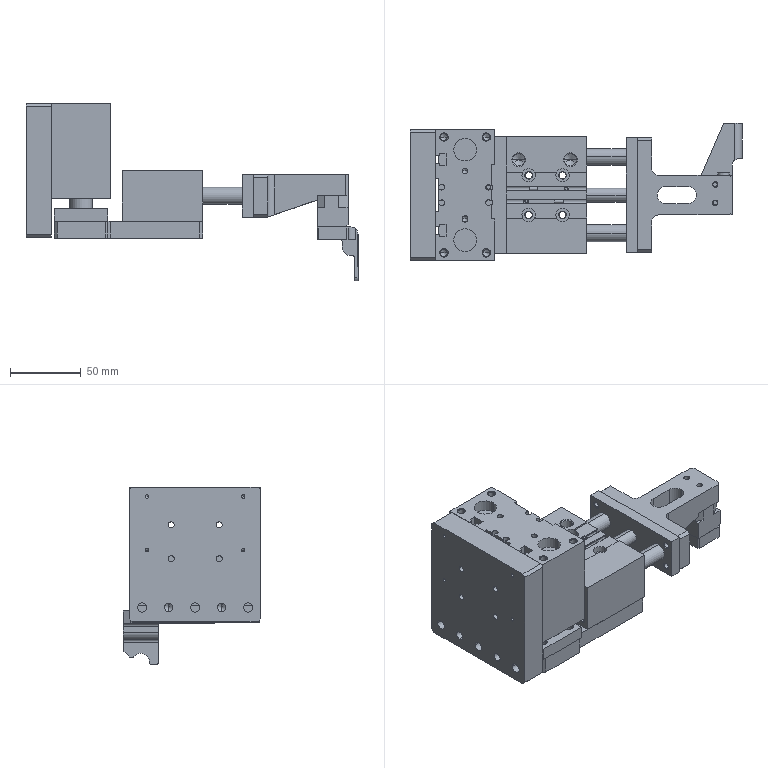Assembly | SolidWorks | mm | 19 component files | 19 solids | 919 faces | box 235 x 97.5 x 125.5 mm | volume 753632 mm3 | cylinder 362 | plane 357 | cone 184 | torus 16 | commonest cylinder face diameters 4 x40 4.917 x32 3 x26 6 x24 8.566 x24 11 x22 6.6 x22 2.5 x16
Bill of materials:
AX.B92.SA.7371.18 | 1 | 6061 | Flat rectangular plate with a wider stepped section at one end, chamfered corners, and a pattern of through holes of three sizes.
AX.B92.SA.7371.20 | 1 | 6061 | T-shaped bracket: a flat arm with an elongated slot and two small holes, joined to a perpendicular mounting flange that has four holes. A tapered web sits under the arm.
AX.B92.SA.7371.25 | 1 | 7075 | Thick square-ish plate with chamfered corners, four small holes in a square pattern, and three larger holes in a row along one edge.
AX.B92.SA.7371.37 | 1 | 40Cr | L-shaped bracket: a flat horizontal arm with two counterbored holes, joined to a downward leg with a rounded outer corner. The leg ends in a semicircular notch.
SCHUNK-0303022 | 2 | 1.231 (40CrMnMoS8-6) | Revolved part with a cylindrical head containing a hexagonal socket, an hourglass-shaped neck groove, a larger cylindrical body, and a smaller end spigot.
D_M9P_MGP_Z_6 | 4 |  | Stepped cylindrical shaft with a smaller pilot end and a long main section that has one wide flat machined along its length.
MGP_Z_PLUG_20_9 | 2 |  | Plain solid cylinder with flat ends and no visible holes, chamfers, or other features.
MGPM20_20Z_0_BODY_2 | 1 |  | Rectangular block with two parallel longitudinal grooves on top, several counterbored or stepped holes, two large cross-bores through the end faces, and T-shaped slots and small round grooves on the bottom.
MGPM20_20Z_0_ROD_4 | 1 |  | Rectangular flange plate with four corner holes and two small central holes, and three parallel round rods sticking out from one face. The middle rod is shorter and has a disc-shaped head.
MGP_Z_PLUG_25_9 | 2 |  | Plain solid cylinder with flat ends and no visible holes, chamfers, or other features. It looks the same as unnamed part.
MGPM25_30Z_0_BODY_2 | 1 |  | Rectangular block with two large vertical through bores, small countersunk holes at the corners, T-shaped slots and semicircular notches along the sides, two parallel vertical grooves on one face, and several side holes.
MGPM25_30Z_0_ROD_4 | 1 |  | Rectangular base plate with four corner holes and three upright cylindrical posts in a row. The middle post is shorter, thinner, and capped with a larger disc.
SCHUNK-0303023 BSWS-B 64 | 1 | Q235-A | Roughly rectangular prismatic block with a stepped, angled notch cut into one vertical corner. Two parallel cylindrical pins with chamfered tips stick up from the top face, and each pin sits in a shallow annular recess. A further short cylindrical boss appears to stick out from a side face that is hidden in the isometric view.
Mates:
1. coincident | AX.B92.SA.7371.25-2 face at (-0.5788, 7.188, 28.472) dir (1, 0, 0) | MGPM25-30Z-M9P-1/MGPM25_30Z_0_BODY_2-1 face at (-0.5788, 65.688, 123.472) dir (-1, 0, 0)
2. width | MGPM25-30Z-M9P-1/MGPM25_30Z_0_BODY_2-1 face at (-0.5788, 100.188, 123.472) dir (0, 1, 0) | MGPM25-30Z-M9P-1/MGPM25_30Z_0_BODY_2-1 face at (41.421, 7.188, 123.472) dir (0, -1, 0) | AX.B92.SA.7371.25-2 face at (-9.579, 100.188, 75.972) dir (0, 1, 0) | AX.B92.SA.7371.25-2 face at (-9.579, 7.188, 75.972) dir (0, -1, 0)
3. coincident | AX.B92.SA.7371.25-2 face at (-0.5788, 7.188, 123.472) dir (0, 0, 1) | MGPM25-30Z-M9P-1/MGPM25_30Z_0_BODY_2-1 face at (36.921, 59.188, 123.472) dir (0, 0, 1)
4. coincident | AX.B92.SA.7371.18-2 face at (53.921, 53.688, 39.972) dir (0, 0, 1) | MGPM25-30Z-M9P-1/MGPM25_30Z_0_ROD_4-1 face at (20.421, 53.688, 39.972) dir (0, 0, -1)
5. concentric | AX.B92.SA.7371.18-2 face at (7.421, 92.688, 27.972) dir (0, 0, -1) r 5.5 | MGPM25-30Z-M9P-1/MGPM25_30Z_0_ROD_4-1 face at (7.421, 92.688, 39.972) dir (0, 0, 1) r 2.458
6. parallel | AX.B92.SA.7371.18-2 face at (106.421, 99.188, 39.972) dir (0, 1, 0) | MGPM25-30Z-M9P-1/MGPM25_30Z_0_ROD_4-1 face at (1.421, 99.188, 48.972) dir (0, 1, 0)
7. concentric | AX.B92.SA.7371.18-2 face at (65.421, 67.688, 27.972) dir (0, 0, -1) r 5.5 | MGPM20-20Z-M9P-1/MGPM20_20Z_0_BODY_2-1 face at (65.421, 67.688, 75.972) dir (0, 0, -1) r 2.458
8. coincident | AX.B92.SA.7371.18-2 face at (53.921, 53.688, 39.972) dir (0, 0, 1) | MGPM20-20Z-M9P-1/MGPM20_20Z_0_BODY_2-1 face at (49.421, 78.388, 39.972) dir (0, 0, -1)
9. parallel | AX.B92.SA.7371.18-2 face at (106.421, 95.188, 39.972) dir (0, 1, 0) | MGPM20-20Z-M9P-1/MGPM20_20Z_0_BODY_2-1 face at (49.421, 95.188, 39.972) dir (0, 1, 0)
10. concentric | MGPM20-20Z-M9P-1/MGPM20_20Z_0_ROD_4-1 face at (142.421, 88.688, 66.972) dir (-1, 0, 0) r 2.067 | AX.B92.SA.7371.20-2 face at (152.421, 88.688, 66.972) dir (1, 0, 0) r 2.75
11. coincident | MGPM20-20Z-M9P-1/MGPM20_20Z_0_ROD_4-1 face at (142.421, 53.688, 57.972) dir (1, 0, 0) | AX.B92.SA.7371.20-2 face at (142.421, 53.688, 57.972) dir (-1, 0, 0)
12. coincident | MGPM20-20Z-M9P-1/MGPM20_20Z_0_ROD_4-1 face at (134.421, 13.188, 42.972) dir (0, 0, -1) | AX.B92.SA.7371.20-2 face at (209.421, 53.688, 42.972) dir (0, 0, -1)
13. coincident | AX.B92.SA.7371.20-2 face at (187.421, 67.688, 57.972) dir (1, 0, 0) | SCHUNK-0303023 BSWS-B 64-1 face at (187.421, 39.688, 57.972) dir (-1, 0, 0)
14. coincident | AX.B92.SA.7371.20-2 face at (209.421, 53.688, 57.972) dir (0, 0, -1) | SCHUNK-0303023 BSWS-B 64-1 face at (209.421, 39.688, 57.972) dir (0, 0, 1)
15. coincident | AX.B92.SA.7371.20-2 face at (209.421, 67.688, 42.972) dir (0, 1, 0) | SCHUNK-0303023 BSWS-B 64-1 face at (197.421, 67.688, 57.972) dir (0, 1, 0)
16. parallel | SCHUNK-0303023 BSWS-B 64-1 face at (187.421, 39.688, 57.972) dir (-1, 0, 0) | GripperA3-2-1/AX.B92.SA.7371.37-1 face at (187.421, 39.688, 35.972) dir (-1, 0, 0)
17. coincident | SCHUNK-0303022-1 face at (197.421, 45.188, 35.972) dir (0, 0, -1) | SCHUNK-0303022-2 face at (197.421, 58.188, 35.972) dir (0, 0, -1)
18. concentric | AX.B92.SA.7371.37-1 face at (197.421, 61.188, 26.972) dir (0, 0, -1) r 4 | SCHUNK-0303022-2 face at (197.421, 61.188, 50.972) dir (0, 0, -1) r 3
19. concentric | AX.B92.SA.7371.37-1 face at (197.421, 48.188, 26.972) dir (0, 0, -1) r 4 | SCHUNK-0303022-1 face at (197.421, 48.188, 50.972) dir (0, 0, -1) r 3
20. coincident | AX.B92.SA.7371.37-1 face at (216.421, 39.688, 35.972) dir (0, 0, 1) | SCHUNK-0303022-1 face at (197.421, 45.188, 35.972) dir (0, 0, -1)
21. distance | MGPM20_20Z_0_ROD_4-1 face at (15, -40.5, 28) dir (1, 0, 0) | MGPM20_20Z_0_BODY_2-1 face at (18, 16.25, -57) dir (1, 0, 0)
22. distance | MGPM20_20Z_0_ROD_4-1 face at (15, 40.5, 28) dir (0, 1, 0) | MGPM20_20Z_0_BODY_2-1 face at (18, 41.5, -57) dir (0, 1, 0)
23. distance | MGPM20_20Z_0_ROD_4-1 face at (0, 0, 28) dir (0, 0, -1) | MGPM20_20Z_0_BODY_2-1 face at (-14.8, 4.45, 0) dir (0, 0, 1)
24. distance | MGPM25_30Z_0_ROD_4-1 face at (19, 45.5, 7) dir (0, 1, 0) | MGPM25_30Z_0_BODY_2-1 face at (21, 46.5, -67.5) dir (0, 1, 0)
25. distance | MGPM25_30Z_0_ROD_4-1 face at (19, -45.5, 7) dir (1, 0, 0) | MGPM25_30Z_0_BODY_2-1 face at (21, 17, -67.5) dir (1, 0, 0)
26. distance | MGPM25_30Z_0_ROD_4-1 face at (0, 0, 16) dir (0, 0, 1) | MGPM25_30Z_0_BODY_2-1 face at (16.5, -5.5, 0) dir (0, 0, 1)